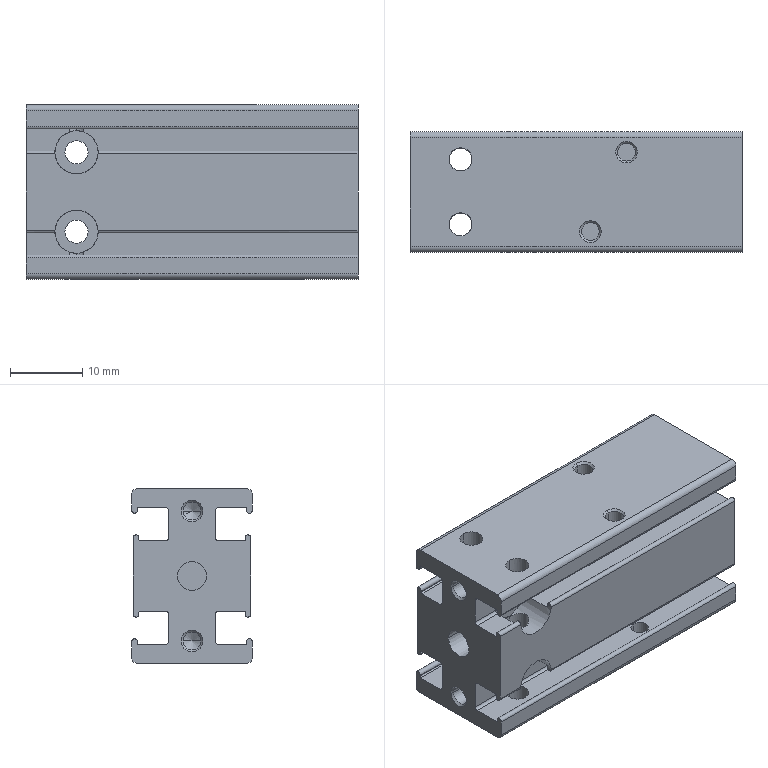Component | SolidWorks | MD-10x10-S-G1-2 (0)-1_MD 10x10-S10 - Body-1 | 1 solid | 194 faces | volume 11213 mm3 | cylinder 124 | plane 42 | cone 28 | commonest cylinder face diameters 0.8 x38 0.4 x18 2.459 x16 3.2 x16 6 x16 4.134 x4 1.6 x4 9 x3